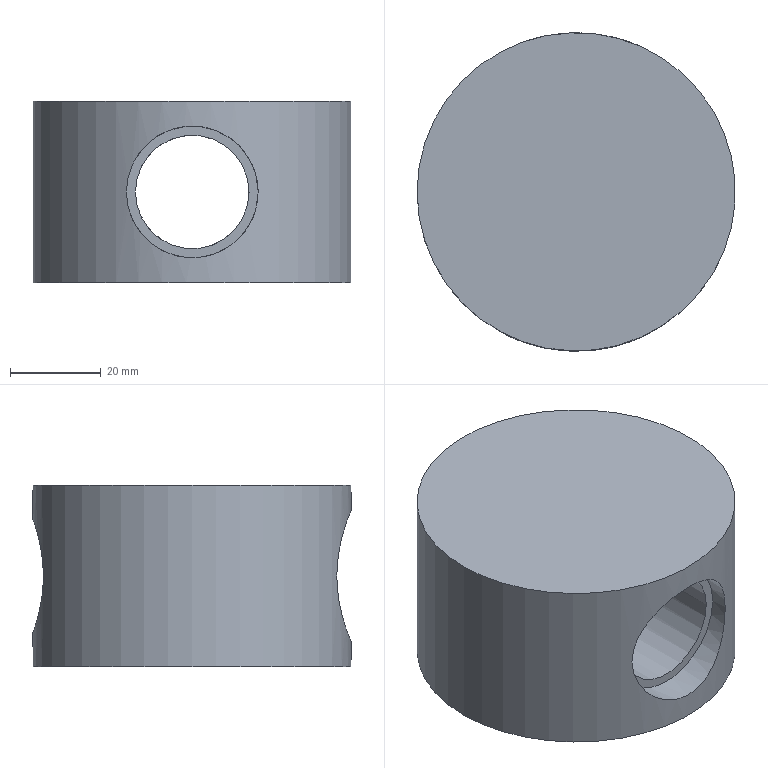Component | NX | 6_DISK | 1 solid | 6 faces | volume 119185 mm3 | plane 3 | cylinder 3 | commonest cylinder face diameters 70 x1 29 x1 25 x1